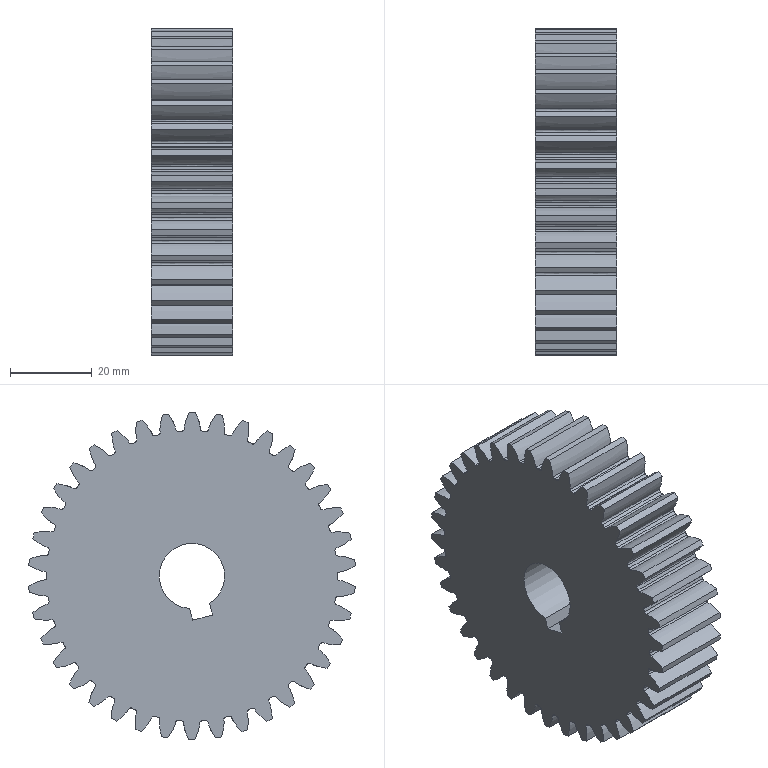Component | NX | CYLINDRICAL_GEAR_38X2 | 1 solid | 234 faces | volume 85672 mm3 | other 190 | cylinder 39 | plane 5 | commonest cylinder face diameters 71 x38 16 x1